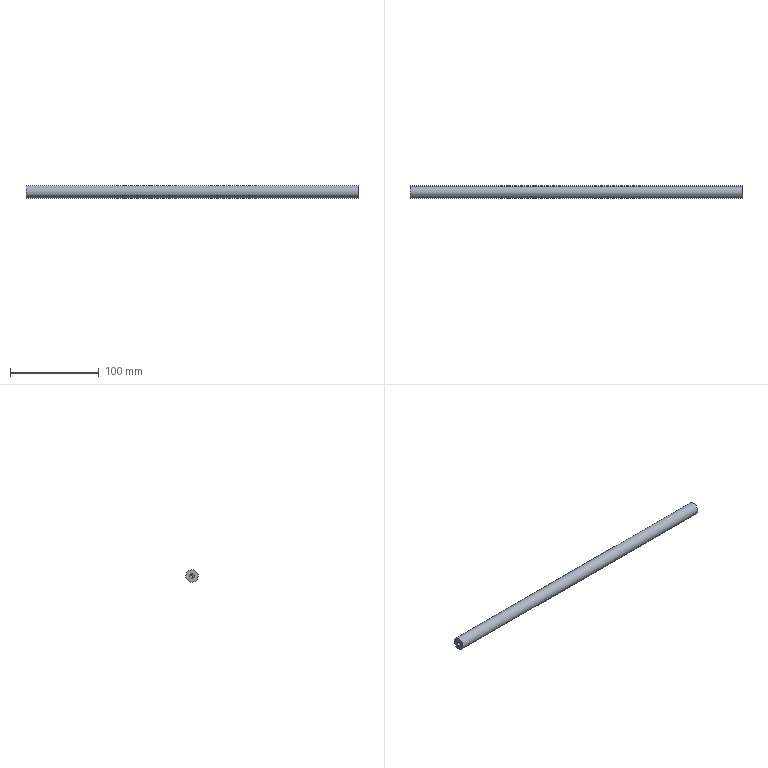Component | SolidWorks | CS021-A10-A006-1 | 1 solid | 12 faces | box 375 x 14 x 14 mm | volume 57040 mm3 | cylinder 6 | cone 4 | plane 2 | commonest cylinder face diameters 5 x4 14 x2 | material AL6061
build123d program:
from build123d import *

# Parameters (mm, degrees)
SKETCH1_R           = 7
BOSS_EXTRUDE1_DEPTH = 187.5


with BuildPart() as part:
    # Sketch1 → Boss-Extrude1 (new, symmetric)
    with BuildSketch(Plane.XY):
        Circle(SKETCH1_R)
    extrude(amount=BOSS_EXTRUDE1_DEPTH, both=True)

    # Sketch2 → M6 Tapped Hole1 (revolve, cut)
    with BuildSketch(Plane(origin=(0, 0, 187.5), x_dir=(0, -1, 0), z_dir=(1, 0, 0))):
        Polygon((0, 0), (0, 18.502), (2.5, 17), (2.5, 0), align=None)
    m6_tapped_hole1 = revolve(axis=Axis((0, 0, 193.85), (0, 0, -1)), mode=Mode.SUBTRACT)

    # Mirror1: M6 Tapped Hole1 across plane
    add(m6_tapped_hole1.mirror(Plane.XY), mode=Mode.SUBTRACT)


solid = part.part

# Placed as in the assembly
solid = solid.moved(Location((33.449, 84.817, -38), (0, 90, 0)))
STEP:
#1=COLOUR_RGB('',0.7922,0.8196,0.9333);
#2=FILL_AREA_STYLE_COLOUR('',#1);
#3=FILL_AREA_STYLE('',(#2));
#4=SURFACE_STYLE_FILL_AREA(#3);
#5=SURFACE_SIDE_STYLE('',(#4));
#6=SURFACE_STYLE_USAGE(.BOTH.,#5);
#7=PRESENTATION_STYLE_ASSIGNMENT((#6));
#8=CARTESIAN_POINT('',(8.029,3.424,-1.446));
#9=VERTEX_POINT('',#8);
#10=CARTESIAN_POINT('',(8.029,3.254,-1.546));
#11=VERTEX_POINT('',#10);
#12=CARTESIAN_POINT('',(8.029,3.339,-1.496));
#13=DIRECTION('',(1.,-0.,-0.));
#14=DIRECTION('',(0.,-0.8617,-0.5074));
#15=AXIS2_PLACEMENT_3D('',#12,#13,#14);
#16=CIRCLE('',#15,0.09843);
#17=EDGE_CURVE('',#9,#11,#16,.T.);
#18=ORIENTED_EDGE('',*,*,#17,.F.);
#19=CARTESIAN_POINT('',(8.699,3.424,-1.446));
#20=VERTEX_POINT('',#19);
#21=CARTESIAN_POINT('',(8.699,3.424,-1.446));
#22=DIRECTION('',(1.,-0.,-0.));
#23=VECTOR('',#22,39.37);
#24=LINE('',#21,#23);
#25=EDGE_CURVE('',#9,#20,#24,.T.);
#26=ORIENTED_EDGE('',*,*,#25,.T.);
#27=CARTESIAN_POINT('',(8.699,3.254,-1.546));
#28=VERTEX_POINT('',#27);
#29=CARTESIAN_POINT('',(8.699,3.339,-1.496));
#30=DIRECTION('',(1.,-0.,-0.));
#31=DIRECTION('',(0.,-0.8617,-0.5074));
#32=AXIS2_PLACEMENT_3D('',#29,#30,#31);
#33=CIRCLE('',#32,0.09843);
#34=EDGE_CURVE('',#20,#28,#33,.T.);
#35=ORIENTED_EDGE('',*,*,#34,.T.);
#36=CARTESIAN_POINT('',(8.699,3.254,-1.546));
#37=DIRECTION('',(1.,-0.,-0.));
#38=VECTOR('',#37,39.37);
#39=LINE('',#36,#38);
#40=EDGE_CURVE('',#11,#28,#39,.T.);
#41=ORIENTED_EDGE('',*,*,#40,.F.);
#42=EDGE_LOOP('',(#18,#26,#35,#41));
#43=FACE_OUTER_BOUND('',#42,.T.);
#44=CARTESIAN_POINT('',(8.699,3.339,-1.496));
#45=DIRECTION('',(1.,-0.,-0.));
#46=DIRECTION('',(0.,-0.8617,-0.5074));
#47=AXIS2_PLACEMENT_3D('',#44,#45,#46);
#48=CYLINDRICAL_SURFACE('',#47,0.09843);
#49=ADVANCED_FACE('',(#43),#48,.F.);
#50=CARTESIAN_POINT('',(7.97,3.339,-1.496));
#51=VERTEX_POINT('',#50);
#52=CARTESIAN_POINT('',(8.029,3.254,-1.546));
#53=DIRECTION('',(0.515,-0.7386,-0.4349));
#54=VECTOR('',#53,39.37);
#55=LINE('',#52,#54);
#56=EDGE_CURVE('',#51,#11,#55,.T.);
#57=ORIENTED_EDGE('',*,*,#56,.F.);
#58=CARTESIAN_POINT('',(8.029,3.424,-1.446));
#59=DIRECTION('',(0.515,0.7386,0.4349));
#60=VECTOR('',#59,39.37);
#61=LINE('',#58,#60);
#62=EDGE_CURVE('',#51,#9,#61,.T.);
#63=ORIENTED_EDGE('',*,*,#62,.T.);
#64=ORIENTED_EDGE('',*,*,#17,.T.);
#65=EDGE_LOOP('',(#57,#63,#64));
#66=FACE_OUTER_BOUND('',#65,.T.);
#67=CARTESIAN_POINT('',(8.029,3.339,-1.496));
#68=DIRECTION('',(1.,-0.,-0.));
#69=DIRECTION('',(0.,-0.8617,-0.5074));
#70=AXIS2_PLACEMENT_3D('',#67,#68,#69);
#71=CONICAL_SURFACE('',#70,0.09843,1.03);
#72=ADVANCED_FACE('',(#66),#71,.F.);
#73=CARTESIAN_POINT('',(-5.396,3.254,-1.546));
#74=VERTEX_POINT('',#73);
#75=CARTESIAN_POINT('',(-5.396,3.424,-1.446));
#76=VERTEX_POINT('',#75);
#77=CARTESIAN_POINT('',(-5.396,3.339,-1.496));
#78=DIRECTION('',(-1.,0.,0.));
#79=DIRECTION('',(0.,0.8617,0.5074));
#80=AXIS2_PLACEMENT_3D('',#77,#78,#79);
#81=CIRCLE('',#80,0.09843);
#82=EDGE_CURVE('',#74,#76,#81,.T.);
#83=ORIENTED_EDGE('',*,*,#82,.F.);
#84=CARTESIAN_POINT('',(-6.065,3.254,-1.546));
#85=VERTEX_POINT('',#84);
#86=CARTESIAN_POINT('',(-6.065,3.254,-1.546));
#87=DIRECTION('',(-1.,0.,0.));
#88=VECTOR('',#87,39.37);
#89=LINE('',#86,#88);
#90=EDGE_CURVE('',#74,#85,#89,.T.);
#91=ORIENTED_EDGE('',*,*,#90,.T.);
#92=CARTESIAN_POINT('',(-6.065,3.424,-1.446));
#93=VERTEX_POINT('',#92);
#94=CARTESIAN_POINT('',(-6.065,3.339,-1.496));
#95=DIRECTION('',(-1.,0.,0.));
#96=DIRECTION('',(0.,0.8617,0.5074));
#97=AXIS2_PLACEMENT_3D('',#94,#95,#96);
#98=CIRCLE('',#97,0.09843);
#99=EDGE_CURVE('',#85,#93,#98,.T.);
#100=ORIENTED_EDGE('',*,*,#99,.T.);
#101=CARTESIAN_POINT('',(-6.065,3.424,-1.446));
#102=DIRECTION('',(-1.,0.,0.));
#103=VECTOR('',#102,39.37);
#104=LINE('',#101,#103);
#105=EDGE_CURVE('',#76,#93,#104,.T.);
#106=ORIENTED_EDGE('',*,*,#105,.F.);
#107=EDGE_LOOP('',(#83,#91,#100,#106));
#108=FACE_OUTER_BOUND('',#107,.T.);
#109=CARTESIAN_POINT('',(-6.065,3.339,-1.496));
#110=DIRECTION('',(-1.,0.,0.));
#111=DIRECTION('',(0.,0.8617,0.5074));
#112=AXIS2_PLACEMENT_3D('',#109,#110,#111);
#113=CYLINDRICAL_SURFACE('',#112,0.09843);
#114=ADVANCED_FACE('',(#108),#113,.F.);
#115=CARTESIAN_POINT('',(-5.337,3.339,-1.496));
#116=VERTEX_POINT('',#115);
#117=CARTESIAN_POINT('',(-5.396,3.424,-1.446));
#118=DIRECTION('',(-0.515,0.7386,0.4349));
#119=VECTOR('',#118,39.37);
#120=LINE('',#117,#119);
#121=EDGE_CURVE('',#116,#76,#120,.T.);
#122=ORIENTED_EDGE('',*,*,#121,.F.);
#123=CARTESIAN_POINT('',(-5.396,3.254,-1.546));
#124=DIRECTION('',(-0.515,-0.7386,-0.4349));
#125=VECTOR('',#124,39.37);
#126=LINE('',#123,#125);
#127=EDGE_CURVE('',#116,#74,#126,.T.);
#128=ORIENTED_EDGE('',*,*,#127,.T.);
#129=ORIENTED_EDGE('',*,*,#82,.T.);
#130=EDGE_LOOP('',(#122,#128,#129));
#131=FACE_OUTER_BOUND('',#130,.T.);
#132=CARTESIAN_POINT('',(-5.396,3.339,-1.496));
#133=DIRECTION('',(-1.,0.,0.));
#134=DIRECTION('',(0.,0.8617,0.5074));
#135=AXIS2_PLACEMENT_3D('',#132,#133,#134);
#136=CONICAL_SURFACE('',#135,0.09843,1.03);
#137=ADVANCED_FACE('',(#131),#136,.F.);
#138=CARTESIAN_POINT('',(-6.065,3.577,-1.356));
#139=VERTEX_POINT('',#138);
#140=CARTESIAN_POINT('',(-6.065,3.102,-1.636));
#141=VERTEX_POINT('',#140);
#142=CARTESIAN_POINT('',(-6.065,3.339,-1.496));
#143=DIRECTION('',(-1.,0.,0.));
#144=DIRECTION('',(0.,0.8617,0.5074));
#145=AXIS2_PLACEMENT_3D('',#142,#143,#144);
#146=CIRCLE('',#145,0.2756);
#147=EDGE_CURVE('',#139,#141,#146,.T.);
#148=ORIENTED_EDGE('',*,*,#147,.F.);
#149=CARTESIAN_POINT('',(8.699,3.577,-1.356));
#150=VERTEX_POINT('',#149);
#151=CARTESIAN_POINT('',(-6.065,3.577,-1.356));
#152=DIRECTION('',(1.,-0.,-0.));
#153=VECTOR('',#152,39.37);
#154=LINE('',#151,#153);
#155=EDGE_CURVE('',#139,#150,#154,.T.);
#156=ORIENTED_EDGE('',*,*,#155,.T.);
#157=CARTESIAN_POINT('',(8.699,3.102,-1.636));
#158=VERTEX_POINT('',#157);
#159=CARTESIAN_POINT('',(8.699,3.339,-1.496));
#160=DIRECTION('',(-1.,0.,0.));
#161=DIRECTION('',(0.,0.8617,0.5074));
#162=AXIS2_PLACEMENT_3D('',#159,#160,#161);
#163=CIRCLE('',#162,0.2756);
#164=EDGE_CURVE('',#150,#158,#163,.T.);
#165=ORIENTED_EDGE('',*,*,#164,.T.);
#166=CARTESIAN_POINT('',(-6.065,3.102,-1.636));
#167=DIRECTION('',(1.,-0.,-0.));
#168=VECTOR('',#167,39.37);
#169=LINE('',#166,#168);
#170=EDGE_CURVE('',#141,#158,#169,.T.);
#171=ORIENTED_EDGE('',*,*,#170,.F.);
#172=EDGE_LOOP('',(#148,#156,#165,#171));
#173=FACE_OUTER_BOUND('',#172,.T.);
#174=CARTESIAN_POINT('',(-6.065,3.339,-1.496));
#175=DIRECTION('',(1.,-0.,-0.));
#176=DIRECTION('',(0.,-0.8617,-0.5074));
#177=AXIS2_PLACEMENT_3D('',#174,#175,#176);
#178=CYLINDRICAL_SURFACE('',#177,0.2756);
#179=ADVANCED_FACE('',(#173),#178,.T.);
#180=ORIENTED_EDGE('',*,*,#155,.F.);
#181=CARTESIAN_POINT('',(-6.065,3.339,-1.496));
#182=DIRECTION('',(-1.,0.,0.));
#183=DIRECTION('',(0.,0.8617,0.5074));
#184=AXIS2_PLACEMENT_3D('',#181,#182,#183);
#185=CIRCLE('',#184,0.2756);
#186=EDGE_CURVE('',#141,#139,#185,.T.);
#187=ORIENTED_EDGE('',*,*,#186,.F.);
#188=ORIENTED_EDGE('',*,*,#170,.T.);
#189=CARTESIAN_POINT('',(8.699,3.339,-1.496));
#190=DIRECTION('',(-1.,0.,0.));
#191=DIRECTION('',(0.,0.8617,0.5074));
#192=AXIS2_PLACEMENT_3D('',#189,#190,#191);
#193=CIRCLE('',#192,0.2756);
#194=EDGE_CURVE('',#158,#150,#193,.T.);
#195=ORIENTED_EDGE('',*,*,#194,.T.);
#196=EDGE_LOOP('',(#180,#187,#188,#195));
#197=FACE_OUTER_BOUND('',#196,.T.);
#198=CARTESIAN_POINT('',(-6.065,3.339,-1.496));
#199=DIRECTION('',(1.,-0.,-0.));
#200=DIRECTION('',(0.,-0.8617,-0.5074));
#201=AXIS2_PLACEMENT_3D('',#198,#199,#200);
#202=CYLINDRICAL_SURFACE('',#201,0.2756);
#203=ADVANCED_FACE('',(#197),#202,.T.);
#204=CARTESIAN_POINT('',(-6.065,3.339,-1.496));
#205=DIRECTION('',(-1.,0.,0.));
#206=DIRECTION('',(0.,0.8617,0.5074));
#207=AXIS2_PLACEMENT_3D('',#204,#205,#206);
#208=CIRCLE('',#207,0.09843);
#209=EDGE_CURVE('',#93,#85,#208,.T.);
#210=ORIENTED_EDGE('',*,*,#209,.F.);
#211=ORIENTED_EDGE('',*,*,#99,.F.);
#212=EDGE_LOOP('',(#210,#211));
#213=FACE_BOUND('',#212,.T.);
#214=ORIENTED_EDGE('',*,*,#186,.T.);
#215=ORIENTED_EDGE('',*,*,#147,.T.);
#216=EDGE_LOOP('',(#214,#215));
#217=FACE_OUTER_BOUND('',#216,.T.);
#218=CARTESIAN_POINT('',(-6.065,3.339,-1.496));
#219=DIRECTION('',(-1.,0.,0.));
#220=DIRECTION('',(0.,0.8617,0.5074));
#221=AXIS2_PLACEMENT_3D('',#218,#219,#220);
#222=PLANE('',#221);
#223=ADVANCED_FACE('',(#213,#217),#222,.T.);
#224=CARTESIAN_POINT('',(8.699,3.339,-1.496));
#225=DIRECTION('',(1.,-0.,-0.));
#226=DIRECTION('',(0.,-0.8617,-0.5074));
#227=AXIS2_PLACEMENT_3D('',#224,#225,#226);
#228=CIRCLE('',#227,0.09843);
#229=EDGE_CURVE('',#28,#20,#228,.T.);
#230=ORIENTED_EDGE('',*,*,#229,.F.);
#231=ORIENTED_EDGE('',*,*,#34,.F.);
#232=EDGE_LOOP('',(#230,#231));
#233=FACE_BOUND('',#232,.T.);
#234=ORIENTED_EDGE('',*,*,#194,.F.);
#235=ORIENTED_EDGE('',*,*,#164,.F.);
#236=EDGE_LOOP('',(#234,#235));
#237=FACE_OUTER_BOUND('',#236,.T.);
#238=CARTESIAN_POINT('',(8.699,3.339,-1.496));
#239=DIRECTION('',(-1.,0.,0.));
#240=DIRECTION('',(0.,0.8617,0.5074));
#241=AXIS2_PLACEMENT_3D('',#238,#239,#240);
#242=PLANE('',#241);
#243=ADVANCED_FACE('',(#233,#237),#242,.F.);
#244=ORIENTED_EDGE('',*,*,#127,.F.);
#245=ORIENTED_EDGE('',*,*,#121,.T.);
#246=CARTESIAN_POINT('',(-5.396,3.339,-1.496));
#247=DIRECTION('',(-1.,0.,0.));
#248=DIRECTION('',(0.,0.8617,0.5074));
#249=AXIS2_PLACEMENT_3D('',#246,#247,#248);
#250=CIRCLE('',#249,0.09843);
#251=EDGE_CURVE('',#76,#74,#250,.T.);
#252=ORIENTED_EDGE('',*,*,#251,.T.);
#253=EDGE_LOOP('',(#244,#245,#252));
#254=FACE_OUTER_BOUND('',#253,.T.);
#255=CARTESIAN_POINT('',(-5.396,3.339,-1.496));
#256=DIRECTION('',(-1.,0.,0.));
#257=DIRECTION('',(0.,0.8617,0.5074));
#258=AXIS2_PLACEMENT_3D('',#255,#256,#257);
#259=CONICAL_SURFACE('',#258,0.09843,1.03);
#260=ADVANCED_FACE('',(#254),#259,.F.);
#261=ORIENTED_EDGE('',*,*,#90,.F.);
#262=ORIENTED_EDGE('',*,*,#251,.F.);
#263=ORIENTED_EDGE('',*,*,#105,.T.);
#264=ORIENTED_EDGE('',*,*,#209,.T.);
#265=EDGE_LOOP('',(#261,#262,#263,#264));
#266=FACE_OUTER_BOUND('',#265,.T.);
#267=CARTESIAN_POINT('',(-6.065,3.339,-1.496));
#268=DIRECTION('',(-1.,0.,0.));
#269=DIRECTION('',(0.,0.8617,0.5074));
#270=AXIS2_PLACEMENT_3D('',#267,#268,#269);
#271=CYLINDRICAL_SURFACE('',#270,0.09843);
#272=ADVANCED_FACE('',(#266),#271,.F.);
#273=ORIENTED_EDGE('',*,*,#62,.F.);
#274=ORIENTED_EDGE('',*,*,#56,.T.);
#275=CARTESIAN_POINT('',(8.029,3.339,-1.496));
#276=DIRECTION('',(1.,-0.,-0.));
#277=DIRECTION('',(0.,-0.8617,-0.5074));
#278=AXIS2_PLACEMENT_3D('',#275,#276,#277);
#279=CIRCLE('',#278,0.09843);
#280=EDGE_CURVE('',#11,#9,#279,.T.);
#281=ORIENTED_EDGE('',*,*,#280,.T.);
#282=EDGE_LOOP('',(#273,#274,#281));
#283=FACE_OUTER_BOUND('',#282,.T.);
#284=CARTESIAN_POINT('',(8.029,3.339,-1.496));
#285=DIRECTION('',(1.,-0.,-0.));
#286=DIRECTION('',(0.,-0.8617,-0.5074));
#287=AXIS2_PLACEMENT_3D('',#284,#285,#286);
#288=CONICAL_SURFACE('',#287,0.09843,1.03);
#289=ADVANCED_FACE('',(#283),#288,.F.);
#290=ORIENTED_EDGE('',*,*,#25,.F.);
#291=ORIENTED_EDGE('',*,*,#280,.F.);
#292=ORIENTED_EDGE('',*,*,#40,.T.);
#293=ORIENTED_EDGE('',*,*,#229,.T.);
#294=EDGE_LOOP('',(#290,#291,#292,#293));
#295=FACE_OUTER_BOUND('',#294,.T.);
#296=CARTESIAN_POINT('',(8.699,3.339,-1.496));
#297=DIRECTION('',(1.,-0.,-0.));
#298=DIRECTION('',(0.,-0.8617,-0.5074));
#299=AXIS2_PLACEMENT_3D('',#296,#297,#298);
#300=CYLINDRICAL_SURFACE('',#299,0.09843);
#301=ADVANCED_FACE('',(#295),#300,.F.);
#302=CLOSED_SHELL('',(#49,#72,#114,#137,#179,#203,#223,#243,#260,#272,#289,#301));
#303=MANIFOLD_SOLID_BREP('',#302);
#304=STYLED_ITEM('',(#7),#303);
#305=(LENGTH_UNIT()NAMED_UNIT(*)SI_UNIT($,.METRE.));
#306=LENGTH_MEASURE_WITH_UNIT(LENGTH_MEASURE(0.0254),#305);
#307=DIMENSIONAL_EXPONENTS(1.,0.,0.,0.,0.,0.,0.);
#308=(CONVERSION_BASED_UNIT('',#306)LENGTH_UNIT()NAMED_UNIT(#307));
#309=UNCERTAINTY_MEASURE_WITH_UNIT(LENGTH_MEASURE(0.00001),#308,'','');
#310=(NAMED_UNIT(*)PLANE_ANGLE_UNIT()SI_UNIT($,.RADIAN.));
#311=(NAMED_UNIT(*)SI_UNIT($,.STERADIAN.)SOLID_ANGLE_UNIT());
#312=(GEOMETRIC_REPRESENTATION_CONTEXT(3)GLOBAL_UNCERTAINTY_ASSIGNED_CONTEXT((#309))GLOBAL_UNIT_ASSIGNED_CONTEXT((#308,#310,#311))REPRESENTATION_CONTEXT('',''));
#313=MECHANICAL_DESIGN_GEOMETRIC_PRESENTATION_REPRESENTATION('',(#304),#312);
#314=CARTESIAN_POINT('',(0.,0.,0.));
#315=DIRECTION('',(0.,0.,1.));
#316=DIRECTION('',(1.,0.,0.));
#317=AXIS2_PLACEMENT_3D('',#314,#315,#316);
#318=(LENGTH_UNIT()NAMED_UNIT(*)SI_UNIT($,.METRE.));
#319=LENGTH_MEASURE_WITH_UNIT(LENGTH_MEASURE(0.0254),#318);
#320=DIMENSIONAL_EXPONENTS(1.,0.,0.,0.,0.,0.,0.);
#321=(CONVERSION_BASED_UNIT('',#319)LENGTH_UNIT()NAMED_UNIT(#320));
#322=UNCERTAINTY_MEASURE_WITH_UNIT(LENGTH_MEASURE(0.00001),#321,'','');
#323=(NAMED_UNIT(*)PLANE_ANGLE_UNIT()SI_UNIT($,.RADIAN.));
#324=(NAMED_UNIT(*)SI_UNIT($,.STERADIAN.)SOLID_ANGLE_UNIT());
#325=(GEOMETRIC_REPRESENTATION_CONTEXT(3)GLOBAL_UNCERTAINTY_ASSIGNED_CONTEXT((#322))GLOBAL_UNIT_ASSIGNED_CONTEXT((#321,#323,#324))REPRESENTATION_CONTEXT('',''));
#326=ADVANCED_BREP_SHAPE_REPRESENTATION('',(#303,#317),#325);
#327=PRESENTATION_LAYER_ASSIGNMENT('','',(#304));